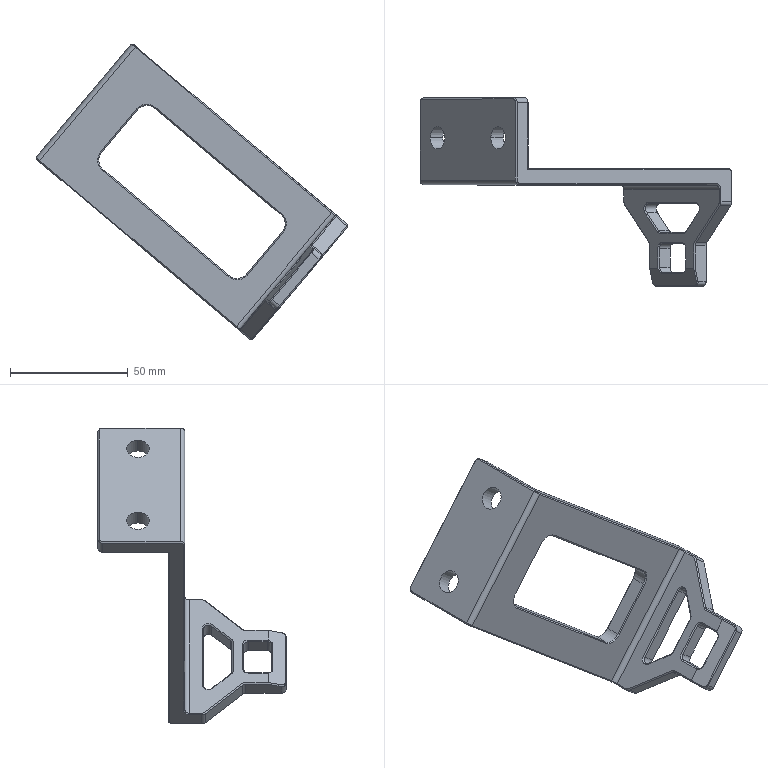Component | SolidWorks | 10GripperJawAA-5 | 1 solid | 154 faces | volume 56021 mm3 | plane 77 | cone 46 | cylinder 27 | spline 4 | commonest cylinder face diameters 4 x19 9.5 x4 10 x4 | material Aviation Aluminum-7075